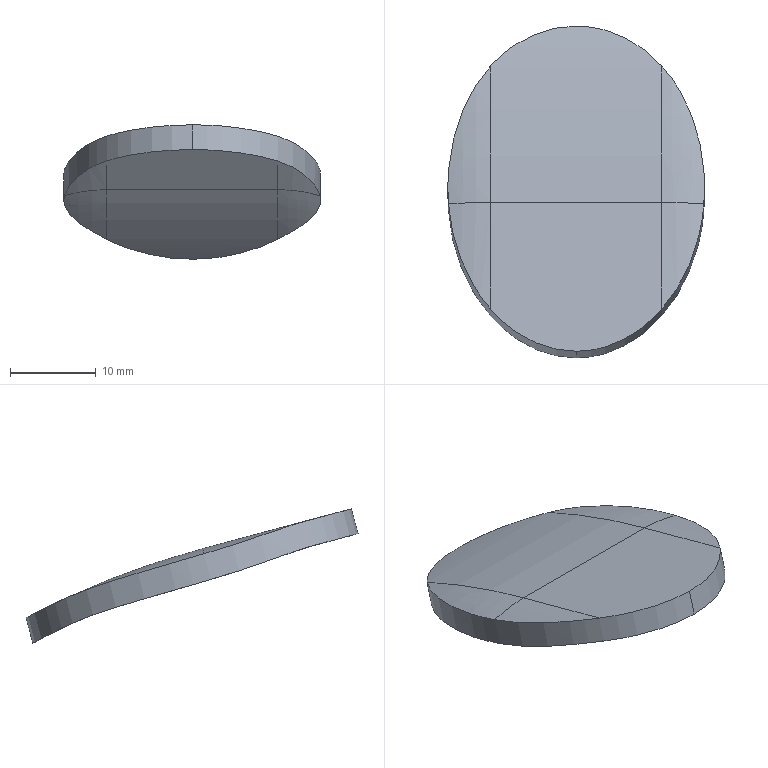Component | SolidWorks | HumanHandle-1_UpperHandle-1_HandleUpperElectrode-1 | 1 solid | 14 faces | box 30 x 38.78 x 15.69 mm | volume 2843 mm3 | cylinder 6 | torus 4 | spline 2 | plane 2 | commonest cylinder face diameters 34 x2 40 x2 194 x1 200 x1 | material Stainless Steel (Ferritic)
STEP:
#1=COLOUR_RGB('',0.7922,0.8196,0.9333);
#2=FILL_AREA_STYLE_COLOUR('',#1);
#3=FILL_AREA_STYLE('',(#2));
#4=SURFACE_STYLE_FILL_AREA(#3);
#5=SURFACE_SIDE_STYLE('',(#4));
#6=SURFACE_STYLE_USAGE(.BOTH.,#5);
#7=PRESENTATION_STYLE_ASSIGNMENT((#6));
#8=CARTESIAN_POINT('',(52.173,58.347,90.88));
#9=VERTEX_POINT('',#8);
#10=CARTESIAN_POINT('',(51.779,58.53,90.789));
#11=VERTEX_POINT('',#10);
#12=CARTESIAN_POINT('',(52.173,58.347,90.88));
#13=CARTESIAN_POINT('',(52.148,58.374,90.868));
#14=CARTESIAN_POINT('',(52.122,58.399,90.856));
#15=CARTESIAN_POINT('',(52.078,58.432,90.839));
#16=CARTESIAN_POINT('',(52.063,58.443,90.834));
#17=CARTESIAN_POINT('',(52.031,58.462,90.824));
#18=CARTESIAN_POINT('',(52.015,58.471,90.819));
#19=CARTESIAN_POINT('',(51.965,58.496,90.807));
#20=CARTESIAN_POINT('',(51.929,58.508,90.8));
#21=CARTESIAN_POINT('',(51.874,58.521,90.793));
#22=CARTESIAN_POINT('',(51.855,58.525,90.792));
#23=CARTESIAN_POINT('',(51.817,58.529,90.789));
#24=CARTESIAN_POINT('',(51.798,58.53,90.789));
#25=CARTESIAN_POINT('',(51.779,58.53,90.789));
#26=B_SPLINE_CURVE_WITH_KNOTS('',3,(#12,#13,#14,#15,#16,#17,#18,#19,#20,#21,#22,#23,#24,#25),.UNSPECIFIED.,.F.,.F.,(4,2,2,2,2,2,4),(0.,0.002914,0.004372,0.005829,0.008743,0.0102,0.01166),.UNSPECIFIED.);
#27=EDGE_CURVE('',#9,#11,#26,.T.);
#28=ORIENTED_EDGE('',*,*,#27,.T.);
#29=CARTESIAN_POINT('',(51.779,58.562,90.906));
#30=VERTEX_POINT('',#29);
#31=CARTESIAN_POINT('',(51.779,57.862,88.293));
#32=DIRECTION('',(0.,0.2588,0.9659));
#33=VECTOR('',#32,39.37);
#34=LINE('',#31,#33);
#35=EDGE_CURVE('',#11,#30,#34,.T.);
#36=ORIENTED_EDGE('',*,*,#35,.T.);
#37=CARTESIAN_POINT('',(52.173,58.378,90.996));
#38=VERTEX_POINT('',#37);
#39=CARTESIAN_POINT('',(52.173,58.378,90.996));
#40=CARTESIAN_POINT('',(52.148,58.405,90.984));
#41=CARTESIAN_POINT('',(52.122,58.43,90.972));
#42=CARTESIAN_POINT('',(52.078,58.464,90.955));
#43=CARTESIAN_POINT('',(52.063,58.474,90.95));
#44=CARTESIAN_POINT('',(52.031,58.494,90.941));
#45=CARTESIAN_POINT('',(52.015,58.503,90.936));
#46=CARTESIAN_POINT('',(51.964,58.527,90.924));
#47=CARTESIAN_POINT('',(51.929,58.54,90.917));
#48=CARTESIAN_POINT('',(51.874,58.553,90.91));
#49=CARTESIAN_POINT('',(51.855,58.556,90.909));
#50=CARTESIAN_POINT('',(51.817,58.561,90.906));
#51=CARTESIAN_POINT('',(51.798,58.562,90.906));
#52=CARTESIAN_POINT('',(51.779,58.562,90.906));
#53=B_SPLINE_CURVE_WITH_KNOTS('',3,(#39,#40,#41,#42,#43,#44,#45,#46,#47,#48,#49,#50,#51,#52),.UNSPECIFIED.,.F.,.F.,(4,2,2,2,2,2,4),(0.,0.002913,0.00437,0.005827,0.00874,0.0102,0.01165),.UNSPECIFIED.);
#54=EDGE_CURVE('',#38,#30,#53,.T.);
#55=ORIENTED_EDGE('',*,*,#54,.F.);
#56=CARTESIAN_POINT('',(52.367,57.744,91.199));
#57=VERTEX_POINT('',#56);
#58=CARTESIAN_POINT('',(52.367,57.744,91.199));
#59=CARTESIAN_POINT('',(52.371,57.801,91.183));
#60=CARTESIAN_POINT('',(52.37,57.858,91.167));
#61=CARTESIAN_POINT('',(52.362,57.943,91.142));
#62=CARTESIAN_POINT('',(52.358,57.971,91.134));
#63=CARTESIAN_POINT('',(52.347,58.027,91.117));
#64=CARTESIAN_POINT('',(52.341,58.054,91.109));
#65=CARTESIAN_POINT('',(52.325,58.109,91.092));
#66=CARTESIAN_POINT('',(52.316,58.136,91.084));
#67=CARTESIAN_POINT('',(52.295,58.189,91.067));
#68=CARTESIAN_POINT('',(52.283,58.215,91.059));
#69=CARTESIAN_POINT('',(52.256,58.265,91.041));
#70=CARTESIAN_POINT('',(52.241,58.289,91.033));
#71=CARTESIAN_POINT('',(52.209,58.335,91.015));
#72=CARTESIAN_POINT('',(52.192,58.358,91.005));
#73=CARTESIAN_POINT('',(52.173,58.378,90.996));
#74=B_SPLINE_CURVE_WITH_KNOTS('',3,(#58,#59,#60,#61,#62,#63,#64,#65,#66,#67,#68,#69,#70,#71,#72,#73),.UNSPECIFIED.,.F.,.F.,(4,2,2,2,2,2,2,4),(0.,0.004509,0.006764,0.009019,0.01127,0.01353,0.01578,0.01804),.UNSPECIFIED.);
#75=EDGE_CURVE('',#57,#38,#74,.T.);
#76=ORIENTED_EDGE('',*,*,#75,.F.);
#77=CARTESIAN_POINT('',(52.173,57.259,91.354));
#78=VERTEX_POINT('',#77);
#79=CARTESIAN_POINT('',(52.173,57.259,91.354));
#80=CARTESIAN_POINT('',(52.188,57.276,91.35));
#81=CARTESIAN_POINT('',(52.201,57.294,91.345));
#82=CARTESIAN_POINT('',(52.228,57.33,91.334));
#83=CARTESIAN_POINT('',(52.24,57.349,91.327));
#84=CARTESIAN_POINT('',(52.262,57.387,91.315));
#85=CARTESIAN_POINT('',(52.273,57.407,91.308));
#86=CARTESIAN_POINT('',(52.292,57.446,91.295));
#87=CARTESIAN_POINT('',(52.301,57.467,91.288));
#88=CARTESIAN_POINT('',(52.325,57.528,91.267));
#89=CARTESIAN_POINT('',(52.337,57.57,91.253));
#90=CARTESIAN_POINT('',(52.357,57.656,91.226));
#91=CARTESIAN_POINT('',(52.363,57.7,91.212));
#92=CARTESIAN_POINT('',(52.367,57.744,91.199));
#93=B_SPLINE_CURVE_WITH_KNOTS('',3,(#79,#80,#81,#82,#83,#84,#85,#86,#87,#88,#89,#90,#91,#92),.UNSPECIFIED.,.F.,.F.,(4,2,2,2,2,2,4),(0.,0.001755,0.003511,0.005266,0.007022,0.01053,0.01404),.UNSPECIFIED.);
#94=EDGE_CURVE('',#78,#57,#93,.T.);
#95=ORIENTED_EDGE('',*,*,#94,.F.);
#96=CARTESIAN_POINT('',(51.779,57.066,91.406));
#97=VERTEX_POINT('',#96);
#98=CARTESIAN_POINT('',(52.173,57.259,91.354));
#99=CARTESIAN_POINT('',(52.063,57.133,91.388));
#100=CARTESIAN_POINT('',(51.926,57.066,91.406));
#101=CARTESIAN_POINT('',(51.779,57.066,91.406));
#102=(BOUNDED_CURVE()B_SPLINE_CURVE(3,(#98,#99,#100,#101),.UNSPECIFIED.,.F.,.F.)B_SPLINE_CURVE_WITH_KNOTS((4,4),(5.553,6.283),.UNSPECIFIED.)CURVE()GEOMETRIC_REPRESENTATION_ITEM()RATIONAL_B_SPLINE_CURVE((1.,0.9561,0.9561,1.))REPRESENTATION_ITEM(''));
#103=EDGE_CURVE('',#78,#97,#102,.T.);
#104=ORIENTED_EDGE('',*,*,#103,.T.);
#105=CARTESIAN_POINT('',(51.779,57.035,91.292));
#106=VERTEX_POINT('',#105);
#107=CARTESIAN_POINT('',(51.779,56.341,88.701));
#108=DIRECTION('',(0.,0.2588,0.9659));
#109=VECTOR('',#108,39.37);
#110=LINE('',#107,#109);
#111=EDGE_CURVE('',#106,#97,#110,.T.);
#112=ORIENTED_EDGE('',*,*,#111,.F.);
#113=CARTESIAN_POINT('',(52.173,57.229,91.24));
#114=VERTEX_POINT('',#113);
#115=CARTESIAN_POINT('',(52.173,57.229,91.24));
#116=CARTESIAN_POINT('',(52.063,57.103,91.274));
#117=CARTESIAN_POINT('',(51.926,57.035,91.292));
#118=CARTESIAN_POINT('',(51.779,57.035,91.292));
#119=(BOUNDED_CURVE()B_SPLINE_CURVE(3,(#115,#116,#117,#118),.UNSPECIFIED.,.F.,.F.)B_SPLINE_CURVE_WITH_KNOTS((4,4),(5.553,6.283),.UNSPECIFIED.)CURVE()GEOMETRIC_REPRESENTATION_ITEM()RATIONAL_B_SPLINE_CURVE((1.,0.9561,0.9561,1.))REPRESENTATION_ITEM(''));
#120=EDGE_CURVE('',#114,#106,#119,.T.);
#121=ORIENTED_EDGE('',*,*,#120,.F.);
#122=CARTESIAN_POINT('',(52.367,57.712,91.081));
#123=VERTEX_POINT('',#122);
#124=CARTESIAN_POINT('',(52.173,57.229,91.24));
#125=CARTESIAN_POINT('',(52.188,57.246,91.236));
#126=CARTESIAN_POINT('',(52.201,57.263,91.231));
#127=CARTESIAN_POINT('',(52.228,57.3,91.219));
#128=CARTESIAN_POINT('',(52.24,57.318,91.213));
#129=CARTESIAN_POINT('',(52.262,57.356,91.2));
#130=CARTESIAN_POINT('',(52.273,57.376,91.193));
#131=CARTESIAN_POINT('',(52.292,57.415,91.179));
#132=CARTESIAN_POINT('',(52.301,57.435,91.172));
#133=CARTESIAN_POINT('',(52.325,57.497,91.151));
#134=CARTESIAN_POINT('',(52.337,57.539,91.136));
#135=CARTESIAN_POINT('',(52.357,57.624,91.108));
#136=CARTESIAN_POINT('',(52.363,57.668,91.094));
#137=CARTESIAN_POINT('',(52.367,57.712,91.081));
#138=B_SPLINE_CURVE_WITH_KNOTS('',3,(#124,#125,#126,#127,#128,#129,#130,#131,#132,#133,#134,#135,#136,#137),.UNSPECIFIED.,.F.,.F.,(4,2,2,2,2,2,4),(0.,0.001756,0.003512,0.005268,0.007024,0.01054,0.01405),.UNSPECIFIED.);
#139=EDGE_CURVE('',#114,#123,#138,.T.);
#140=ORIENTED_EDGE('',*,*,#139,.T.);
#141=CARTESIAN_POINT('',(52.367,57.712,91.081));
#142=CARTESIAN_POINT('',(52.371,57.769,91.064));
#143=CARTESIAN_POINT('',(52.37,57.826,91.048));
#144=CARTESIAN_POINT('',(52.362,57.911,91.023));
#145=CARTESIAN_POINT('',(52.358,57.939,91.015));
#146=CARTESIAN_POINT('',(52.347,57.995,90.999));
#147=CARTESIAN_POINT('',(52.341,58.023,90.991));
#148=CARTESIAN_POINT('',(52.325,58.078,90.975));
#149=CARTESIAN_POINT('',(52.316,58.105,90.967));
#150=CARTESIAN_POINT('',(52.295,58.158,90.951));
#151=CARTESIAN_POINT('',(52.283,58.183,90.942));
#152=CARTESIAN_POINT('',(52.256,58.234,90.926));
#153=CARTESIAN_POINT('',(52.241,58.258,90.917));
#154=CARTESIAN_POINT('',(52.209,58.305,90.899));
#155=CARTESIAN_POINT('',(52.192,58.327,90.89));
#156=CARTESIAN_POINT('',(52.173,58.347,90.88));
#157=B_SPLINE_CURVE_WITH_KNOTS('',3,(#141,#142,#143,#144,#145,#146,#147,#148,#149,#150,#151,#152,#153,#154,#155,#156),.UNSPECIFIED.,.F.,.F.,(4,2,2,2,2,2,2,4),(0.,0.004509,0.006763,0.009017,0.01127,0.01353,0.01578,0.01803),.UNSPECIFIED.);
#158=EDGE_CURVE('',#123,#9,#157,.T.);
#159=ORIENTED_EDGE('',*,*,#158,.T.);
#160=EDGE_LOOP('',(#28,#36,#55,#76,#95,#104,#112,#121,#140,#159));
#161=FACE_OUTER_BOUND('',#160,.T.);
#162=CARTESIAN_POINT('',(51.779,57.009,91.195));
#163=CARTESIAN_POINT('',(51.779,57.066,91.406));
#164=CARTESIAN_POINT('',(52.96,57.009,91.195));
#165=CARTESIAN_POINT('',(52.96,57.066,91.406));
#166=CARTESIAN_POINT('',(52.96,58.53,90.787));
#167=CARTESIAN_POINT('',(52.96,58.587,90.999));
#168=CARTESIAN_POINT('',(51.779,58.53,90.787));
#169=CARTESIAN_POINT('',(51.779,58.587,90.999));
#170=(BOUNDED_SURFACE()B_SPLINE_SURFACE(3,1,((#162,#163),(#164,#165),(#166,#167),(#168,#169)),.UNSPECIFIED.,.F.,.F.,.F.)B_SPLINE_SURFACE_WITH_KNOTS((4,4),(2,2),(0.,1.),(0.,1.),.UNSPECIFIED.)GEOMETRIC_REPRESENTATION_ITEM()RATIONAL_B_SPLINE_SURFACE(((1.,1.),(0.3333,0.3333),(0.3333,0.3333),(1.,1.)))REPRESENTATION_ITEM('')SURFACE());
#171=ADVANCED_FACE('',(#161),#170,.T.);
#172=CARTESIAN_POINT('',(51.385,58.347,90.88));
#173=VERTEX_POINT('',#172);
#174=CARTESIAN_POINT('',(51.191,57.712,91.081));
#175=VERTEX_POINT('',#174);
#176=CARTESIAN_POINT('',(51.385,58.347,90.88));
#177=CARTESIAN_POINT('',(51.347,58.306,90.9));
#178=CARTESIAN_POINT('',(51.316,58.259,90.917));
#179=CARTESIAN_POINT('',(51.276,58.184,90.942));
#180=CARTESIAN_POINT('',(51.264,58.158,90.95));
#181=CARTESIAN_POINT('',(51.243,58.105,90.967));
#182=CARTESIAN_POINT('',(51.233,58.078,90.975));
#183=CARTESIAN_POINT('',(51.217,58.023,90.991));
#184=CARTESIAN_POINT('',(51.211,57.996,90.999));
#185=CARTESIAN_POINT('',(51.2,57.94,91.015));
#186=CARTESIAN_POINT('',(51.196,57.911,91.023));
#187=CARTESIAN_POINT('',(51.19,57.855,91.04));
#188=CARTESIAN_POINT('',(51.189,57.826,91.048));
#189=CARTESIAN_POINT('',(51.188,57.769,91.064));
#190=CARTESIAN_POINT('',(51.189,57.741,91.073));
#191=CARTESIAN_POINT('',(51.191,57.712,91.081));
#192=B_SPLINE_CURVE_WITH_KNOTS('',3,(#176,#177,#178,#179,#180,#181,#182,#183,#184,#185,#186,#187,#188,#189,#190,#191),.UNSPECIFIED.,.F.,.F.,(4,2,2,2,2,2,2,4),(0.,0.004484,0.006726,0.008968,0.01121,0.01345,0.01569,0.01794),.UNSPECIFIED.);
#193=EDGE_CURVE('',#173,#175,#192,.T.);
#194=ORIENTED_EDGE('',*,*,#193,.F.);
#195=CARTESIAN_POINT('',(51.385,57.72,91.109));
#196=VERTEX_POINT('',#195);
#197=CARTESIAN_POINT('',(51.385,56.731,87.42));
#198=DIRECTION('',(1.,-0.,-0.));
#199=DIRECTION('',(-0.,-0.9659,0.2588));
#200=AXIS2_PLACEMENT_3D('',#197,#198,#199);
#201=CIRCLE('',#200,3.819);
#202=EDGE_CURVE('',#173,#196,#201,.T.);
#203=ORIENTED_EDGE('',*,*,#202,.T.);
#204=CARTESIAN_POINT('',(51.385,57.546,90.462));
#205=DIRECTION('',(0.,0.9659,-0.2588));
#206=DIRECTION('',(-0.,-0.2588,-0.9659));
#207=AXIS2_PLACEMENT_3D('',#204,#205,#206);
#208=CIRCLE('',#207,0.6693);
#209=EDGE_CURVE('',#175,#196,#208,.T.);
#210=ORIENTED_EDGE('',*,*,#209,.F.);
#211=EDGE_LOOP('',(#194,#203,#210));
#212=FACE_OUTER_BOUND('',#211,.T.);
#213=CARTESIAN_POINT('',(51.385,56.731,87.42));
#214=DIRECTION('',(-1.,0.,0.));
#215=DIRECTION('',(-0.,-0.9659,0.2588));
#216=AXIS2_PLACEMENT_3D('',#213,#214,#215);
#217=TOROIDAL_SURFACE('',#216,3.15,0.6693);
#218=ADVANCED_FACE('',(#212),#217,.F.);
#219=CARTESIAN_POINT('',(51.385,57.229,91.24));
#220=VERTEX_POINT('',#219);
#221=CARTESIAN_POINT('',(51.191,57.712,91.081));
#222=CARTESIAN_POINT('',(51.195,57.668,91.094));
#223=CARTESIAN_POINT('',(51.201,57.624,91.108));
#224=CARTESIAN_POINT('',(51.216,57.56,91.129));
#225=CARTESIAN_POINT('',(51.221,57.539,91.136));
#226=CARTESIAN_POINT('',(51.234,57.497,91.151));
#227=CARTESIAN_POINT('',(51.241,57.476,91.158));
#228=CARTESIAN_POINT('',(51.257,57.436,91.172));
#229=CARTESIAN_POINT('',(51.266,57.415,91.179));
#230=CARTESIAN_POINT('',(51.285,57.376,91.193));
#231=CARTESIAN_POINT('',(51.296,57.356,91.2));
#232=CARTESIAN_POINT('',(51.318,57.318,91.213));
#233=CARTESIAN_POINT('',(51.33,57.3,91.219));
#234=CARTESIAN_POINT('',(51.357,57.263,91.231));
#235=CARTESIAN_POINT('',(51.37,57.246,91.236));
#236=CARTESIAN_POINT('',(51.385,57.229,91.24));
#237=B_SPLINE_CURVE_WITH_KNOTS('',3,(#221,#222,#223,#224,#225,#226,#227,#228,#229,#230,#231,#232,#233,#234,#235,#236),.UNSPECIFIED.,.F.,.F.,(4,2,2,2,2,2,2,4),(0.,0.003509,0.005263,0.007017,0.008772,0.01053,0.01228,0.01403),.UNSPECIFIED.);
#238=EDGE_CURVE('',#175,#220,#237,.T.);
#239=ORIENTED_EDGE('',*,*,#238,.F.);
#240=ORIENTED_EDGE('',*,*,#209,.T.);
#241=CARTESIAN_POINT('',(51.385,51.282,92.834));
#242=DIRECTION('',(-0.,-0.9659,0.2588));
#243=VECTOR('',#242,39.37);
#244=LINE('',#241,#243);
#245=EDGE_CURVE('',#196,#220,#244,.T.);
#246=ORIENTED_EDGE('',*,*,#245,.T.);
#247=EDGE_LOOP('',(#239,#240,#246));
#248=FACE_OUTER_BOUND('',#247,.T.);
#249=CARTESIAN_POINT('',(51.385,51.109,92.187));
#250=DIRECTION('',(0.,0.9659,-0.2588));
#251=DIRECTION('',(-1.,0.,0.));
#252=AXIS2_PLACEMENT_3D('',#249,#250,#251);
#253=CYLINDRICAL_SURFACE('',#252,0.6693);
#254=ADVANCED_FACE('',(#248),#253,.F.);
#255=ORIENTED_EDGE('',*,*,#158,.F.);
#256=CARTESIAN_POINT('',(52.173,57.72,91.109));
#257=VERTEX_POINT('',#256);
#258=CARTESIAN_POINT('',(52.173,57.546,90.462));
#259=DIRECTION('',(0.,0.9659,-0.2588));
#260=DIRECTION('',(-0.,-0.2588,-0.9659));
#261=AXIS2_PLACEMENT_3D('',#258,#259,#260);
#262=CIRCLE('',#261,0.6693);
#263=EDGE_CURVE('',#257,#123,#262,.T.);
#264=ORIENTED_EDGE('',*,*,#263,.F.);
#265=CARTESIAN_POINT('',(52.173,56.731,87.42));
#266=DIRECTION('',(-1.,0.,0.));
#267=DIRECTION('',(-0.,-0.9659,0.2588));
#268=AXIS2_PLACEMENT_3D('',#265,#266,#267);
#269=CIRCLE('',#268,3.819);
#270=EDGE_CURVE('',#257,#9,#269,.T.);
#271=ORIENTED_EDGE('',*,*,#270,.T.);
#272=EDGE_LOOP('',(#255,#264,#271));
#273=FACE_OUTER_BOUND('',#272,.T.);
#274=CARTESIAN_POINT('',(52.173,56.731,87.42));
#275=DIRECTION('',(-1.,0.,0.));
#276=DIRECTION('',(-0.,-0.9659,0.2588));
#277=AXIS2_PLACEMENT_3D('',#274,#275,#276);
#278=TOROIDAL_SURFACE('',#277,3.15,0.6693);
#279=ADVANCED_FACE('',(#273),#278,.F.);
#280=ORIENTED_EDGE('',*,*,#139,.F.);
#281=CARTESIAN_POINT('',(52.173,51.282,92.834));
#282=DIRECTION('',(0.,0.9659,-0.2588));
#283=VECTOR('',#282,39.37);
#284=LINE('',#281,#283);
#285=EDGE_CURVE('',#114,#257,#284,.T.);
#286=ORIENTED_EDGE('',*,*,#285,.T.);
#287=ORIENTED_EDGE('',*,*,#263,.T.);
#288=EDGE_LOOP('',(#280,#286,#287));
#289=FACE_OUTER_BOUND('',#288,.T.);
#290=CARTESIAN_POINT('',(52.173,51.109,92.187));
#291=DIRECTION('',(-0.,-0.9659,0.2588));
#292=DIRECTION('',(1.,-0.,0.));
#293=AXIS2_PLACEMENT_3D('',#290,#291,#292);
#294=CYLINDRICAL_SURFACE('',#293,0.6693);
#295=ADVANCED_FACE('',(#289),#294,.F.);
#296=ORIENTED_EDGE('',*,*,#27,.F.);
#297=ORIENTED_EDGE('',*,*,#270,.F.);
#298=CARTESIAN_POINT('',(52.96,57.72,91.109));
#299=DIRECTION('',(-1.,0.,0.));
#300=VECTOR('',#299,39.37);
#301=LINE('',#298,#300);
#302=EDGE_CURVE('',#257,#196,#301,.T.);
#303=ORIENTED_EDGE('',*,*,#302,.T.);
#304=ORIENTED_EDGE('',*,*,#202,.F.);
#305=CARTESIAN_POINT('',(51.779,58.53,90.789));
#306=CARTESIAN_POINT('',(51.74,58.53,90.789));
#307=CARTESIAN_POINT('',(51.703,58.526,90.791));
#308=CARTESIAN_POINT('',(51.647,58.513,90.798));
#309=CARTESIAN_POINT('',(51.629,58.507,90.801));
#310=CARTESIAN_POINT('',(51.594,58.495,90.807));
#311=CARTESIAN_POINT('',(51.576,58.487,90.811));
#312=CARTESIAN_POINT('',(51.526,58.463,90.824));
#313=CARTESIAN_POINT('',(51.494,58.443,90.834));
#314=CARTESIAN_POINT('',(51.436,58.399,90.856));
#315=CARTESIAN_POINT('',(51.41,58.374,90.868));
#316=CARTESIAN_POINT('',(51.385,58.347,90.88));
#317=B_SPLINE_CURVE_WITH_KNOTS('',3,(#305,#306,#307,#308,#309,#310,#311,#312,#313,#314,#315,#316),.UNSPECIFIED.,.F.,.F.,(4,2,2,2,2,4),(0.01166,0.01458,0.01604,0.0175,0.02042,0.02334),.UNSPECIFIED.);
#318=EDGE_CURVE('',#11,#173,#317,.T.);
#319=ORIENTED_EDGE('',*,*,#318,.F.);
#320=EDGE_LOOP('',(#296,#297,#303,#304,#319));
#321=FACE_OUTER_BOUND('',#320,.T.);
#322=CARTESIAN_POINT('',(52.96,56.731,87.42));
#323=DIRECTION('',(-1.,0.,0.));
#324=DIRECTION('',(-0.,-0.9659,0.2588));
#325=AXIS2_PLACEMENT_3D('',#322,#323,#324);
#326=CYLINDRICAL_SURFACE('',#325,3.819);
#327=ADVANCED_FACE('',(#321),#326,.F.);
#328=ORIENTED_EDGE('',*,*,#285,.F.);
#329=ORIENTED_EDGE('',*,*,#120,.T.);
#330=CARTESIAN_POINT('',(51.779,57.035,91.292));
#331=CARTESIAN_POINT('',(51.632,57.035,91.292));
#332=CARTESIAN_POINT('',(51.495,57.103,91.274));
#333=CARTESIAN_POINT('',(51.385,57.229,91.24));
#334=(BOUNDED_CURVE()B_SPLINE_CURVE(3,(#330,#331,#332,#333),.UNSPECIFIED.,.F.,.F.)B_SPLINE_CURVE_WITH_KNOTS((4,4),(0.,0.7297),.UNSPECIFIED.)CURVE()GEOMETRIC_REPRESENTATION_ITEM()RATIONAL_B_SPLINE_CURVE((1.,0.9561,0.9561,1.))REPRESENTATION_ITEM(''));
#335=EDGE_CURVE('',#106,#220,#334,.T.);
#336=ORIENTED_EDGE('',*,*,#335,.T.);
#337=ORIENTED_EDGE('',*,*,#245,.F.);
#338=ORIENTED_EDGE('',*,*,#302,.F.);
#339=EDGE_LOOP('',(#328,#329,#336,#337,#338));
#340=FACE_OUTER_BOUND('',#339,.T.);
#341=CARTESIAN_POINT('',(52.96,51.282,92.834));
#342=DIRECTION('',(-0.,-0.2588,-0.9659));
#343=DIRECTION('',(0.,0.9659,-0.2588));
#344=AXIS2_PLACEMENT_3D('',#341,#342,#343);
#345=PLANE('',#344);
#346=ADVANCED_FACE('',(#340),#345,.T.);
#347=ORIENTED_EDGE('',*,*,#35,.F.);
#348=ORIENTED_EDGE('',*,*,#318,.T.);
#349=ORIENTED_EDGE('',*,*,#193,.T.);
#350=ORIENTED_EDGE('',*,*,#238,.T.);
#351=ORIENTED_EDGE('',*,*,#335,.F.);
#352=ORIENTED_EDGE('',*,*,#111,.T.);
#353=CARTESIAN_POINT('',(51.385,57.259,91.354));
#354=VERTEX_POINT('',#353);
#355=CARTESIAN_POINT('',(51.779,57.066,91.406));
#356=CARTESIAN_POINT('',(51.632,57.066,91.406));
#357=CARTESIAN_POINT('',(51.495,57.133,91.388));
#358=CARTESIAN_POINT('',(51.385,57.259,91.354));
#359=(BOUNDED_CURVE()B_SPLINE_CURVE(3,(#355,#356,#357,#358),.UNSPECIFIED.,.F.,.F.)B_SPLINE_CURVE_WITH_KNOTS((4,4),(0.,0.7297),.UNSPECIFIED.)CURVE()GEOMETRIC_REPRESENTATION_ITEM()RATIONAL_B_SPLINE_CURVE((1.,0.9561,0.9561,1.))REPRESENTATION_ITEM(''));
#360=EDGE_CURVE('',#97,#354,#359,.T.);
#361=ORIENTED_EDGE('',*,*,#360,.T.);
#362=CARTESIAN_POINT('',(51.191,57.744,91.199));
#363=VERTEX_POINT('',#362);
#364=CARTESIAN_POINT('',(51.191,57.744,91.199));
#365=CARTESIAN_POINT('',(51.195,57.7,91.212));
#366=CARTESIAN_POINT('',(51.201,57.656,91.226));
#367=CARTESIAN_POINT('',(51.216,57.592,91.246));
#368=CARTESIAN_POINT('',(51.221,57.57,91.253));
#369=CARTESIAN_POINT('',(51.234,57.528,91.267));
#370=CARTESIAN_POINT('',(51.241,57.508,91.274));
#371=CARTESIAN_POINT('',(51.257,57.467,91.288));
#372=CARTESIAN_POINT('',(51.266,57.446,91.295));
#373=CARTESIAN_POINT('',(51.285,57.407,91.308));
#374=CARTESIAN_POINT('',(51.296,57.387,91.315));
#375=CARTESIAN_POINT('',(51.318,57.349,91.328));
#376=CARTESIAN_POINT('',(51.33,57.33,91.334));
#377=CARTESIAN_POINT('',(51.357,57.294,91.345));
#378=CARTESIAN_POINT('',(51.37,57.276,91.35));
#379=CARTESIAN_POINT('',(51.385,57.259,91.354));
#380=B_SPLINE_CURVE_WITH_KNOTS('',3,(#364,#365,#366,#367,#368,#369,#370,#371,#372,#373,#374,#375,#376,#377,#378,#379),.UNSPECIFIED.,.F.,.F.,(4,2,2,2,2,2,2,4),(0.,0.003507,0.005261,0.007014,0.008768,0.01052,0.01228,0.01403),.UNSPECIFIED.);
#381=EDGE_CURVE('',#363,#354,#380,.T.);
#382=ORIENTED_EDGE('',*,*,#381,.F.);
#383=CARTESIAN_POINT('',(51.385,58.378,90.996));
#384=VERTEX_POINT('',#383);
#385=CARTESIAN_POINT('',(51.385,58.378,90.996));
#386=CARTESIAN_POINT('',(51.347,58.337,91.015));
#387=CARTESIAN_POINT('',(51.316,58.29,91.033));
#388=CARTESIAN_POINT('',(51.276,58.215,91.058));
#389=CARTESIAN_POINT('',(51.264,58.19,91.067));
#390=CARTESIAN_POINT('',(51.243,58.137,91.084));
#391=CARTESIAN_POINT('',(51.233,58.11,91.092));
#392=CARTESIAN_POINT('',(51.217,58.055,91.109));
#393=CARTESIAN_POINT('',(51.211,58.027,91.117));
#394=CARTESIAN_POINT('',(51.2,57.971,91.133));
#395=CARTESIAN_POINT('',(51.196,57.943,91.142));
#396=CARTESIAN_POINT('',(51.19,57.886,91.158));
#397=CARTESIAN_POINT('',(51.189,57.858,91.167));
#398=CARTESIAN_POINT('',(51.188,57.801,91.183));
#399=CARTESIAN_POINT('',(51.189,57.772,91.191));
#400=CARTESIAN_POINT('',(51.191,57.744,91.199));
#401=B_SPLINE_CURVE_WITH_KNOTS('',3,(#385,#386,#387,#388,#389,#390,#391,#392,#393,#394,#395,#396,#397,#398,#399,#400),.UNSPECIFIED.,.F.,.F.,(4,2,2,2,2,2,2,4),(0.,0.004485,0.006728,0.00897,0.01121,0.01346,0.0157,0.01794),.UNSPECIFIED.);
#402=EDGE_CURVE('',#384,#363,#401,.T.);
#403=ORIENTED_EDGE('',*,*,#402,.F.);
#404=CARTESIAN_POINT('',(51.779,58.562,90.906));
#405=CARTESIAN_POINT('',(51.741,58.562,90.906));
#406=CARTESIAN_POINT('',(51.703,58.557,90.908));
#407=CARTESIAN_POINT('',(51.647,58.544,90.915));
#408=CARTESIAN_POINT('',(51.629,58.539,90.918));
#409=CARTESIAN_POINT('',(51.594,58.526,90.924));
#410=CARTESIAN_POINT('',(51.576,58.519,90.928));
#411=CARTESIAN_POINT('',(51.543,58.502,90.936));
#412=CARTESIAN_POINT('',(51.527,58.493,90.941));
#413=CARTESIAN_POINT('',(51.495,58.474,90.95));
#414=CARTESIAN_POINT('',(51.48,58.463,90.956));
#415=CARTESIAN_POINT('',(51.436,58.43,90.972));
#416=CARTESIAN_POINT('',(51.41,58.405,90.983));
#417=CARTESIAN_POINT('',(51.385,58.378,90.996));
#418=B_SPLINE_CURVE_WITH_KNOTS('',3,(#404,#405,#406,#407,#408,#409,#410,#411,#412,#413,#414,#415,#416,#417),.UNSPECIFIED.,.F.,.F.,(4,2,2,2,2,2,4),(0.01165,0.01457,0.01603,0.01749,0.01895,0.02041,0.02333),.UNSPECIFIED.);
#419=EDGE_CURVE('',#30,#384,#418,.T.);
#420=ORIENTED_EDGE('',*,*,#419,.F.);
#421=EDGE_LOOP('',(#347,#348,#349,#350,#351,#352,#361,#382,#403,#420));
#422=FACE_OUTER_BOUND('',#421,.T.);
#423=CARTESIAN_POINT('',(51.779,58.53,90.787));
#424=CARTESIAN_POINT('',(51.779,58.587,90.999));
#425=CARTESIAN_POINT('',(50.598,58.53,90.787));
#426=CARTESIAN_POINT('',(50.598,58.587,90.999));
#427=CARTESIAN_POINT('',(50.598,57.009,91.195));
#428=CARTESIAN_POINT('',(50.598,57.066,91.406));
#429=CARTESIAN_POINT('',(51.779,57.009,91.195));
#430=CARTESIAN_POINT('',(51.779,57.066,91.406));
#431=(BOUNDED_SURFACE()B_SPLINE_SURFACE(3,1,((#423,#424),(#425,#426),(#427,#428),(#429,#430)),.UNSPECIFIED.,.F.,.F.,.F.)B_SPLINE_SURFACE_WITH_KNOTS((4,4),(2,2),(0.,1.),(0.,1.),.UNSPECIFIED.)GEOMETRIC_REPRESENTATION_ITEM()RATIONAL_B_SPLINE_SURFACE(((1.,1.),(0.3333,0.3333),(0.3333,0.3333),(1.,1.)))REPRESENTATION_ITEM('')SURFACE());
#432=ADVANCED_FACE('',(#422),#431,.T.);
#433=ORIENTED_EDGE('',*,*,#103,.F.);
#434=CARTESIAN_POINT('',(52.173,57.75,91.223));
#435=VERTEX_POINT('',#434);
#436=CARTESIAN_POINT('',(52.173,51.313,92.948));
#437=DIRECTION('',(0.,0.9659,-0.2588));
#438=VECTOR('',#437,39.37);
#439=LINE('',#436,#438);
#440=EDGE_CURVE('',#78,#435,#439,.T.);
#441=ORIENTED_EDGE('',*,*,#440,.T.);
#442=CARTESIAN_POINT('',(51.385,57.75,91.223));
#443=VERTEX_POINT('',#442);
#444=CARTESIAN_POINT('',(52.96,57.75,91.223));
#445=DIRECTION('',(-1.,0.,0.));
#446=VECTOR('',#445,39.37);
#447=LINE('',#444,#446);
#448=EDGE_CURVE('',#435,#443,#447,.T.);
#449=ORIENTED_EDGE('',*,*,#448,.T.);
#450=CARTESIAN_POINT('',(51.385,51.313,92.948));
#451=DIRECTION('',(-0.,-0.9659,0.2588));
#452=VECTOR('',#451,39.37);
#453=LINE('',#450,#452);
#454=EDGE_CURVE('',#443,#354,#453,.T.);
#455=ORIENTED_EDGE('',*,*,#454,.T.);
#456=ORIENTED_EDGE('',*,*,#360,.F.);
#457=EDGE_LOOP('',(#433,#441,#449,#455,#456));
#458=FACE_OUTER_BOUND('',#457,.T.);
#459=CARTESIAN_POINT('',(52.96,51.313,92.948));
#460=DIRECTION('',(-0.,-0.2588,-0.9659));
#461=DIRECTION('',(0.,0.9659,-0.2588));
#462=AXIS2_PLACEMENT_3D('',#459,#460,#461);
#463=PLANE('',#462);
#464=ADVANCED_FACE('',(#458),#463,.F.);
#465=CARTESIAN_POINT('',(52.173,56.731,87.42));
#466=DIRECTION('',(-1.,0.,0.));
#467=DIRECTION('',(-0.,-0.9659,0.2588));
#468=AXIS2_PLACEMENT_3D('',#465,#466,#467);
#469=CIRCLE('',#468,3.937);
#470=EDGE_CURVE('',#435,#38,#469,.T.);
#471=ORIENTED_EDGE('',*,*,#470,.T.);
#472=ORIENTED_EDGE('',*,*,#54,.T.);
#473=ORIENTED_EDGE('',*,*,#419,.T.);
#474=CARTESIAN_POINT('',(51.385,56.731,87.42));
#475=DIRECTION('',(1.,-0.,-0.));
#476=DIRECTION('',(-0.,-0.9659,0.2588));
#477=AXIS2_PLACEMENT_3D('',#474,#475,#476);
#478=CIRCLE('',#477,3.937);
#479=EDGE_CURVE('',#384,#443,#478,.T.);
#480=ORIENTED_EDGE('',*,*,#479,.T.);
#481=ORIENTED_EDGE('',*,*,#448,.F.);
#482=EDGE_LOOP('',(#471,#472,#473,#480,#481));
#483=FACE_OUTER_BOUND('',#482,.T.);
#484=CARTESIAN_POINT('',(52.96,56.731,87.42));
#485=DIRECTION('',(-1.,0.,0.));
#486=DIRECTION('',(-0.,-0.9659,0.2588));
#487=AXIS2_PLACEMENT_3D('',#484,#485,#486);
#488=CYLINDRICAL_SURFACE('',#487,3.937);
#489=ADVANCED_FACE('',(#483),#488,.T.);
#490=CARTESIAN_POINT('',(51.385,57.546,90.462));
#491=DIRECTION('',(0.,0.9659,-0.2588));
#492=DIRECTION('',(-1.,0.,0.));
#493=AXIS2_PLACEMENT_3D('',#490,#491,#492);
#494=CIRCLE('',#493,0.7874);
#495=EDGE_CURVE('',#363,#443,#494,.T.);
#496=ORIENTED_EDGE('',*,*,#495,.F.);
#497=ORIENTED_EDGE('',*,*,#381,.T.);
#498=ORIENTED_EDGE('',*,*,#454,.F.);
#499=EDGE_LOOP('',(#496,#497,#498));
#500=FACE_OUTER_BOUND('',#499,.T.);
#501=CARTESIAN_POINT('',(51.385,51.109,92.187));
#502=DIRECTION('',(0.,0.9659,-0.2588));
#503=DIRECTION('',(-1.,0.,0.));
#504=AXIS2_PLACEMENT_3D('',#501,#502,#503);
#505=CYLINDRICAL_SURFACE('',#504,0.7874);
#506=ADVANCED_FACE('',(#500),#505,.T.);
#507=ORIENTED_EDGE('',*,*,#479,.F.);
#508=ORIENTED_EDGE('',*,*,#402,.T.);
#509=ORIENTED_EDGE('',*,*,#495,.T.);
#510=EDGE_LOOP('',(#507,#508,#509));
#511=FACE_OUTER_BOUND('',#510,.T.);
#512=CARTESIAN_POINT('',(51.385,56.731,87.42));
#513=DIRECTION('',(-1.,0.,0.));
#514=DIRECTION('',(-0.,-0.9659,0.2588));
#515=AXIS2_PLACEMENT_3D('',#512,#513,#514);
#516=TOROIDAL_SURFACE('',#515,3.15,0.7874);
#517=ADVANCED_FACE('',(#511),#516,.T.);
#518=ORIENTED_EDGE('',*,*,#440,.F.);
#519=ORIENTED_EDGE('',*,*,#94,.T.);
#520=CARTESIAN_POINT('',(52.173,57.546,90.462));
#521=DIRECTION('',(0.,0.9659,-0.2588));
#522=DIRECTION('',(-1.,0.,0.));
#523=AXIS2_PLACEMENT_3D('',#520,#521,#522);
#524=CIRCLE('',#523,0.7874);
#525=EDGE_CURVE('',#435,#57,#524,.T.);
#526=ORIENTED_EDGE('',*,*,#525,.F.);
#527=EDGE_LOOP('',(#518,#519,#526));
#528=FACE_OUTER_BOUND('',#527,.T.);
#529=CARTESIAN_POINT('',(52.173,51.109,92.187));
#530=DIRECTION('',(-0.,-0.9659,0.2588));
#531=DIRECTION('',(1.,-0.,0.));
#532=AXIS2_PLACEMENT_3D('',#529,#530,#531);
#533=CYLINDRICAL_SURFACE('',#532,0.7874);
#534=ADVANCED_FACE('',(#528),#533,.T.);
#535=ORIENTED_EDGE('',*,*,#525,.T.);
#536=ORIENTED_EDGE('',*,*,#75,.T.);
#537=ORIENTED_EDGE('',*,*,#470,.F.);
#538=EDGE_LOOP('',(#535,#536,#537));
#539=FACE_OUTER_BOUND('',#538,.T.);
#540=CARTESIAN_POINT('',(52.173,56.731,87.42));
#541=DIRECTION('',(-1.,0.,0.));
#542=DIRECTION('',(-0.,-0.9659,0.2588));
#543=AXIS2_PLACEMENT_3D('',#540,#541,#542);
#544=TOROIDAL_SURFACE('',#543,3.15,0.7874);
#545=ADVANCED_FACE('',(#539),#544,.T.);
#546=CLOSED_SHELL('',(#171,#218,#254,#279,#295,#327,#346,#432,#464,#489,#506,#517,#534,#545));
#547=MANIFOLD_SOLID_BREP('',#546);
#548=STYLED_ITEM('',(#7),#547);
#549=PRESENTATION_LAYER_ASSIGNMENT('','',(#548));
#550=(LENGTH_UNIT()NAMED_UNIT(*)SI_UNIT($,.METRE.));
#551=LENGTH_MEASURE_WITH_UNIT(LENGTH_MEASURE(0.0254),#550);
#552=DIMENSIONAL_EXPONENTS(1.,0.,0.,0.,0.,0.,0.);
#553=(CONVERSION_BASED_UNIT('',#551)LENGTH_UNIT()NAMED_UNIT(#552));
#554=UNCERTAINTY_MEASURE_WITH_UNIT(LENGTH_MEASURE(0.00001),#553,'','');
#555=(NAMED_UNIT(*)PLANE_ANGLE_UNIT()SI_UNIT($,.RADIAN.));
#556=(NAMED_UNIT(*)SI_UNIT($,.STERADIAN.)SOLID_ANGLE_UNIT());
#557=(GEOMETRIC_REPRESENTATION_CONTEXT(3)GLOBAL_UNCERTAINTY_ASSIGNED_CONTEXT((#554))GLOBAL_UNIT_ASSIGNED_CONTEXT((#553,#555,#556))REPRESENTATION_CONTEXT('',''));
#558=MECHANICAL_DESIGN_GEOMETRIC_PRESENTATION_REPRESENTATION('',(#548),#557);
#559=CARTESIAN_POINT('',(0.,0.,0.));
#560=DIRECTION('',(0.,0.,1.));
#561=DIRECTION('',(1.,0.,0.));
#562=AXIS2_PLACEMENT_3D('',#559,#560,#561);
#563=(LENGTH_UNIT()NAMED_UNIT(*)SI_UNIT($,.METRE.));
#564=LENGTH_MEASURE_WITH_UNIT(LENGTH_MEASURE(0.0254),#563);
#565=DIMENSIONAL_EXPONENTS(1.,0.,0.,0.,0.,0.,0.);
#566=(CONVERSION_BASED_UNIT('',#564)LENGTH_UNIT()NAMED_UNIT(#565));
#567=UNCERTAINTY_MEASURE_WITH_UNIT(LENGTH_MEASURE(0.00001),#566,'','');
#568=(NAMED_UNIT(*)PLANE_ANGLE_UNIT()SI_UNIT($,.RADIAN.));
#569=(NAMED_UNIT(*)SI_UNIT($,.STERADIAN.)SOLID_ANGLE_UNIT());
#570=(GEOMETRIC_REPRESENTATION_CONTEXT(3)GLOBAL_UNCERTAINTY_ASSIGNED_CONTEXT((#567))GLOBAL_UNIT_ASSIGNED_CONTEXT((#566,#568,#569))REPRESENTATION_CONTEXT('',''));
#571=ADVANCED_BREP_SHAPE_REPRESENTATION('',(#547,#562),#570);